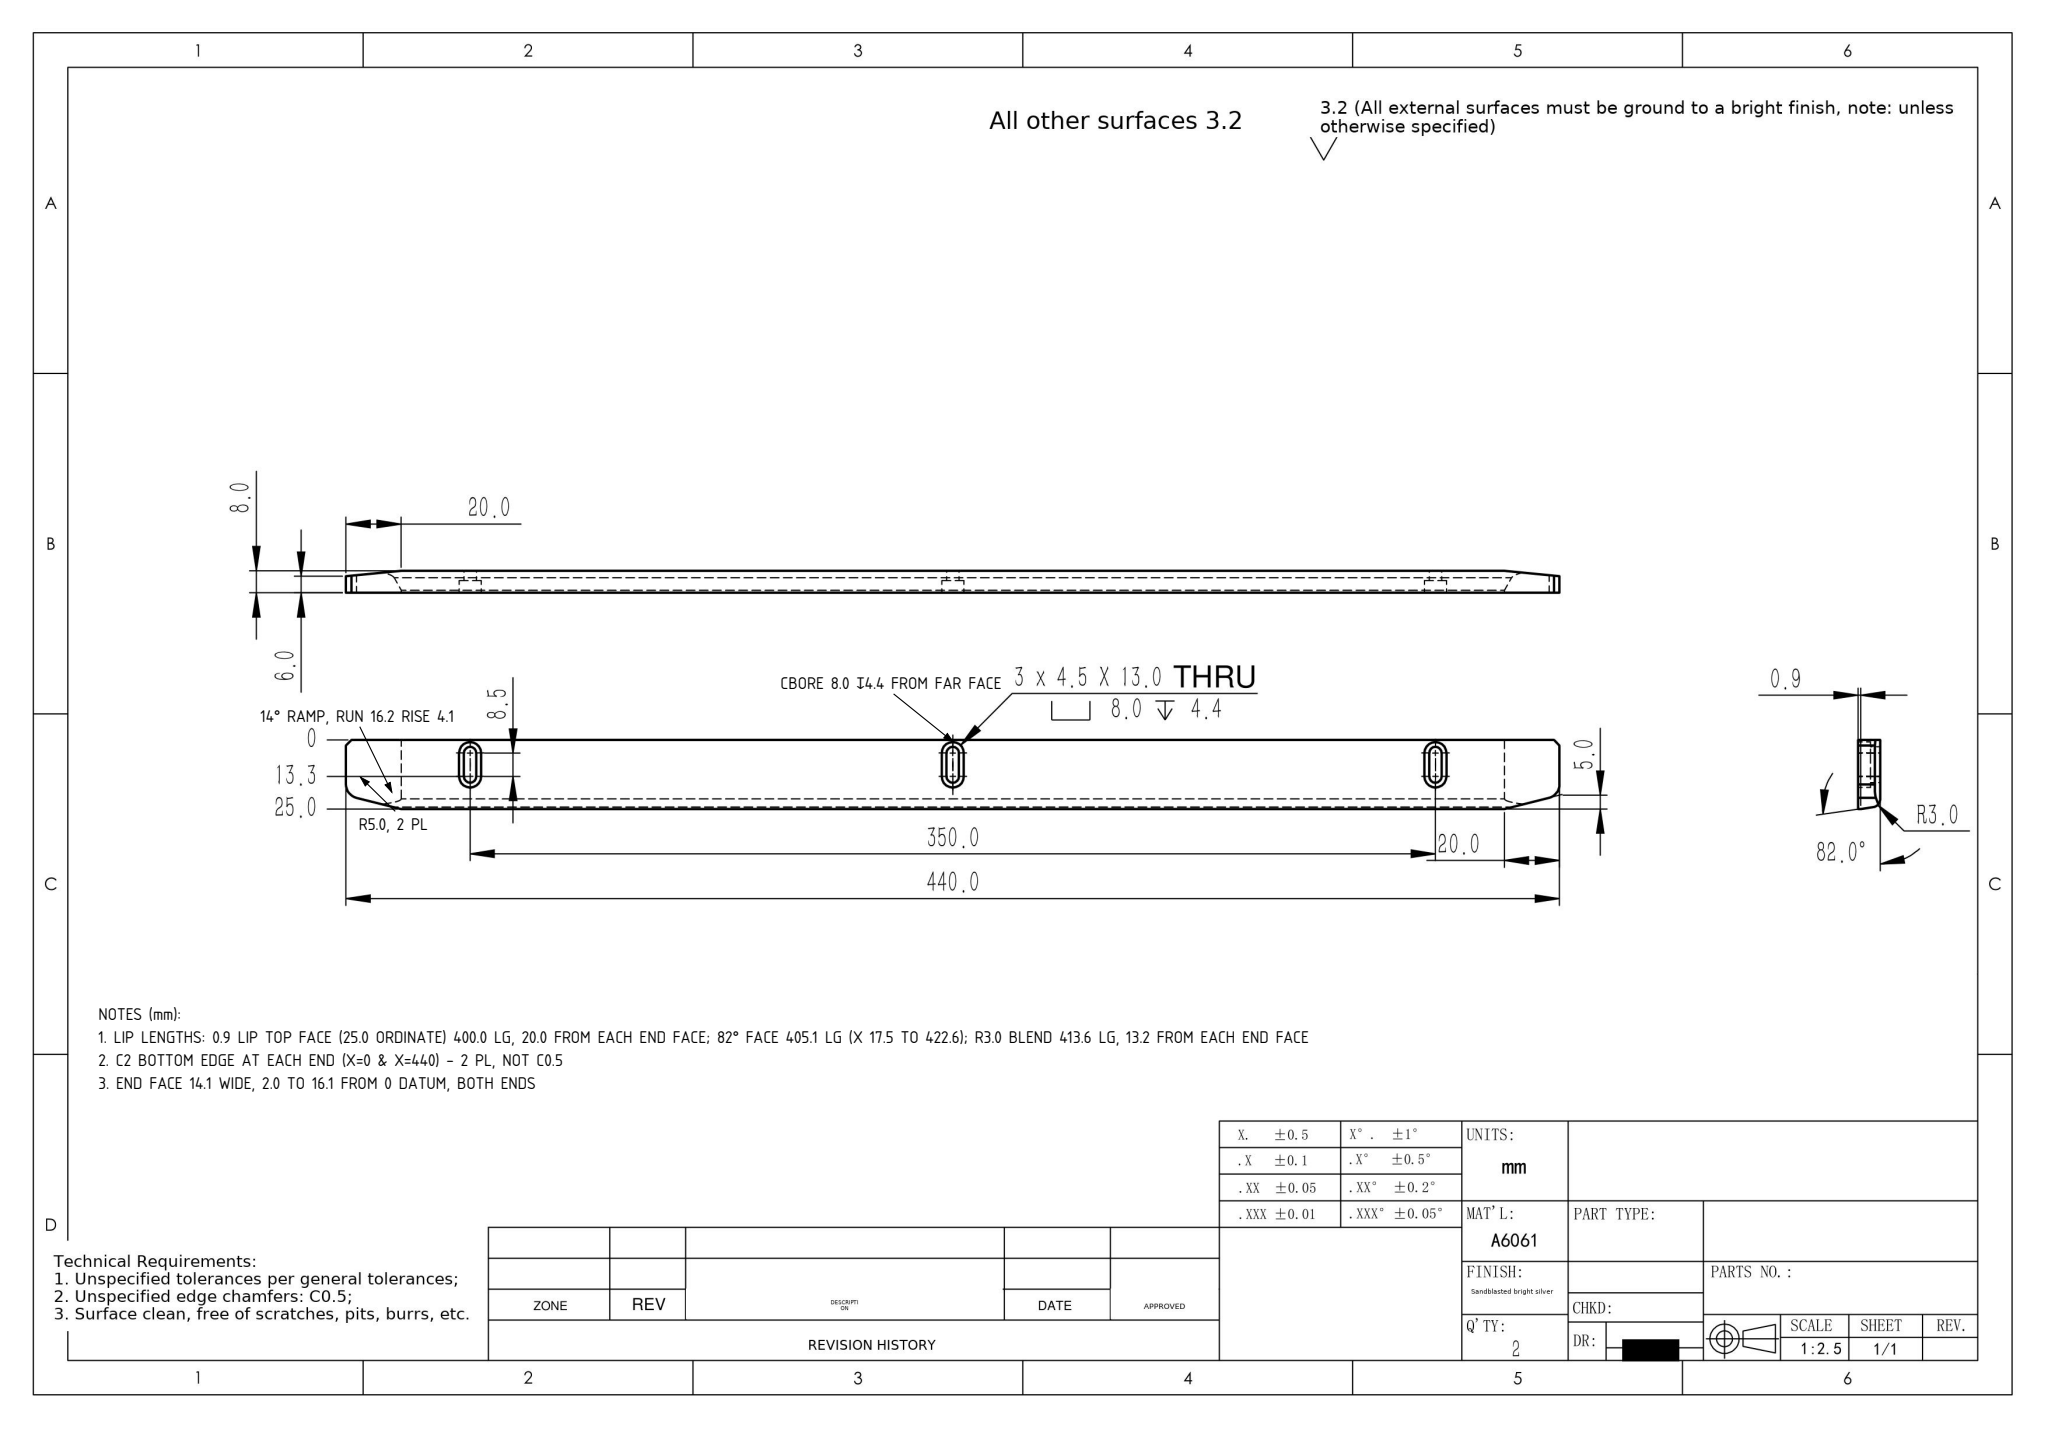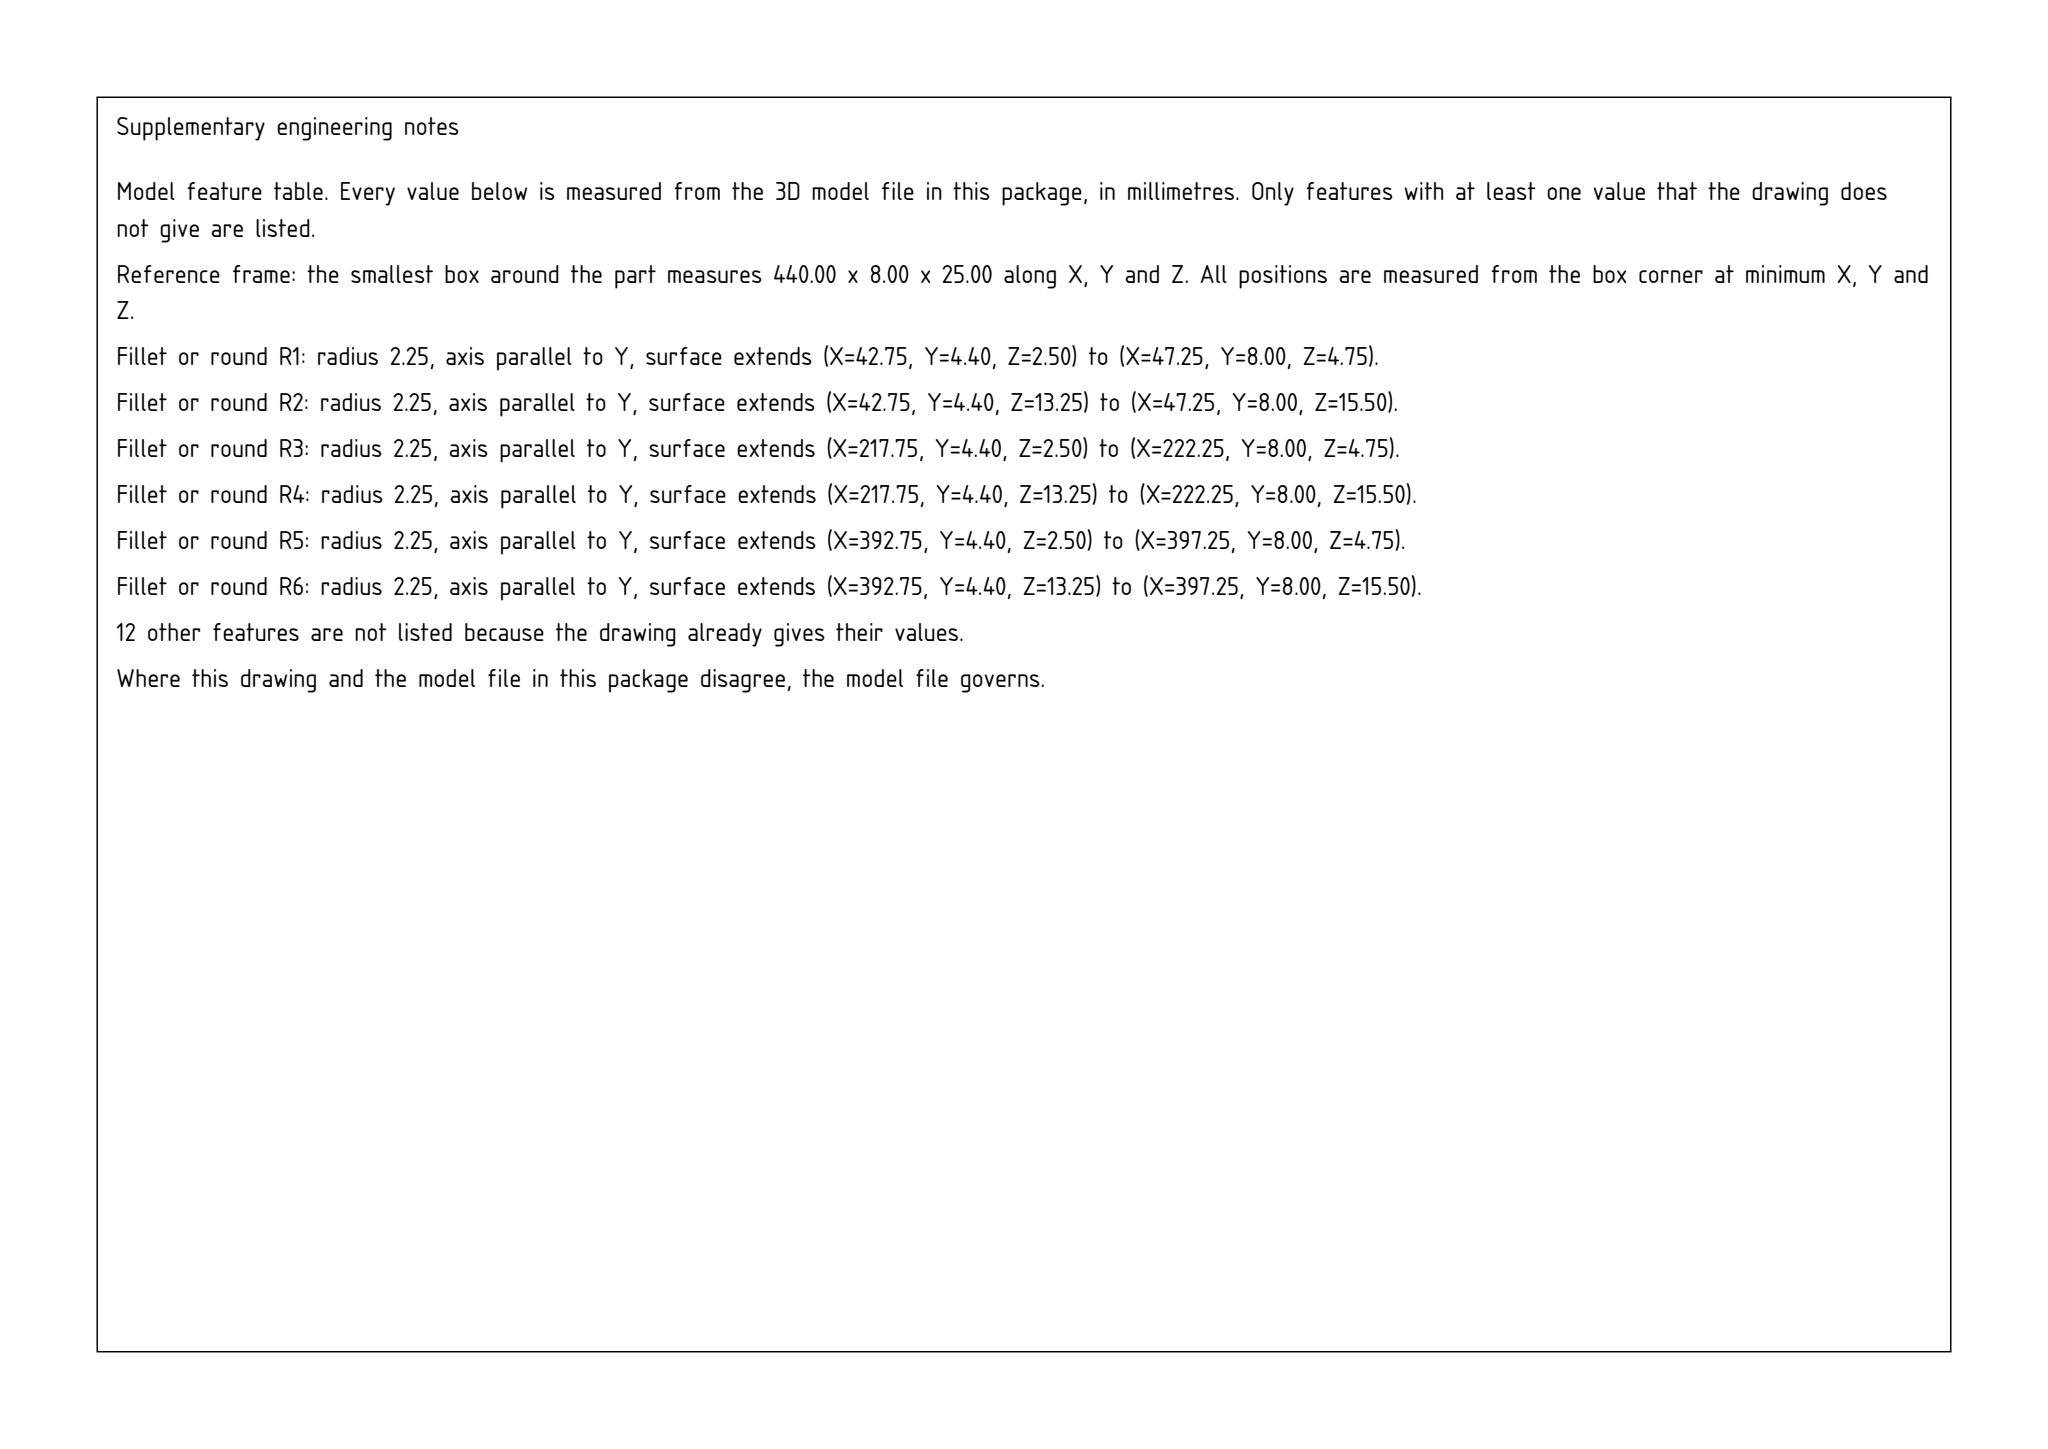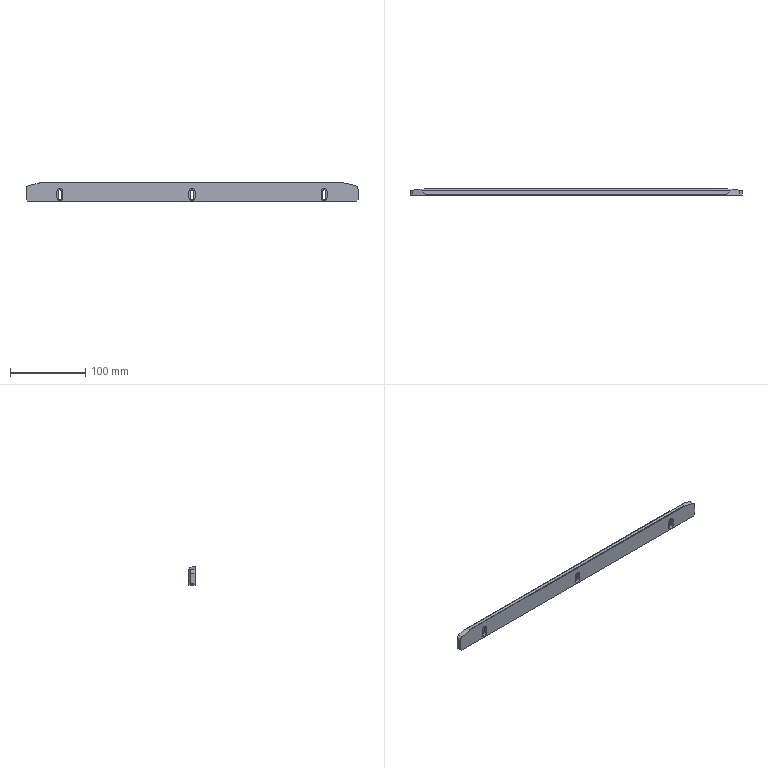Part | SolidWorks | mm | material A6061 | 1 solid | 49 faces | box 440 x 8 x 25 mm | volume 82133 mm3 | plane 28 | cylinder 21 | commonest cylinder face diameters 8 x9 4.5 x9 10 x2 6 x1
Drawing notes:
LIP LENGTHS: 0.9 LIP TOP FACE (25.0 ORDINATE) 400.0 LG, 20.0 FROM EACH END FACE; 82° FACE 405.1 LG (X 17.5 TO 422.6); R3.0 BLEND 413.6 LG, 13.2 FROM EACH END FACE | from the solid: z=25.0 plane extent x [20.0, 420.0] (400.0 long, 20.0 in from each end face of the 440.0 bbox); inclined 82° plane bbox_from [17.5, 0.9, 24.4] size [405.1, 4.5, 0.6]; convex arc dia 6.0 (R3.0) about x axis at (y 5.0, z 21.4) from x 13.2 to 426.8 = 413.6 long
3X SLOT: C'BORE 8.0 WIDE DP 4.4 FROM FULL FLAT FACE (Y=0 SIDE) | from the solid: Dia 8.0 arcs run y 0.0 to 4.4; dia 4.5 arcs y 4.4 to 8.0; y=0 plane is full 440x25 flat face
C2 BOTTOM EDGE AT EACH END (X=0 & X=440) - 2 PL, NOT C0.5 | from the solid: inclined_planes 45/90/45 at bbox_from [0,0,0] and [438,0,0], size 2.0 x 2.0
PLAN VIEW END RAMP 14° FROM 25.0 FACE AT 20.0, RUN 16.2 RISE 4.1 | from the solid: inclined_planes 76/90/14, bbox_from [3.8,0,20.9] & [420,0,20.9], size 16.2 x 4.1
R5.0 END CORNER, CTR 5.0 FROM END & 16.1 FROM 0 DATUM, 2 PL | from the solid: convex arc dia 10.0 axis y at [5.0,-,16.1] and [435.0,-,16.1], 76 deg
END FACE 14.1 WIDE, 2.0 TO 16.1 FROM 0 DATUM, BOTH ENDS | from the solid: axis_planes x=0.0 and x=440.0, extent z [2.0,16.1]